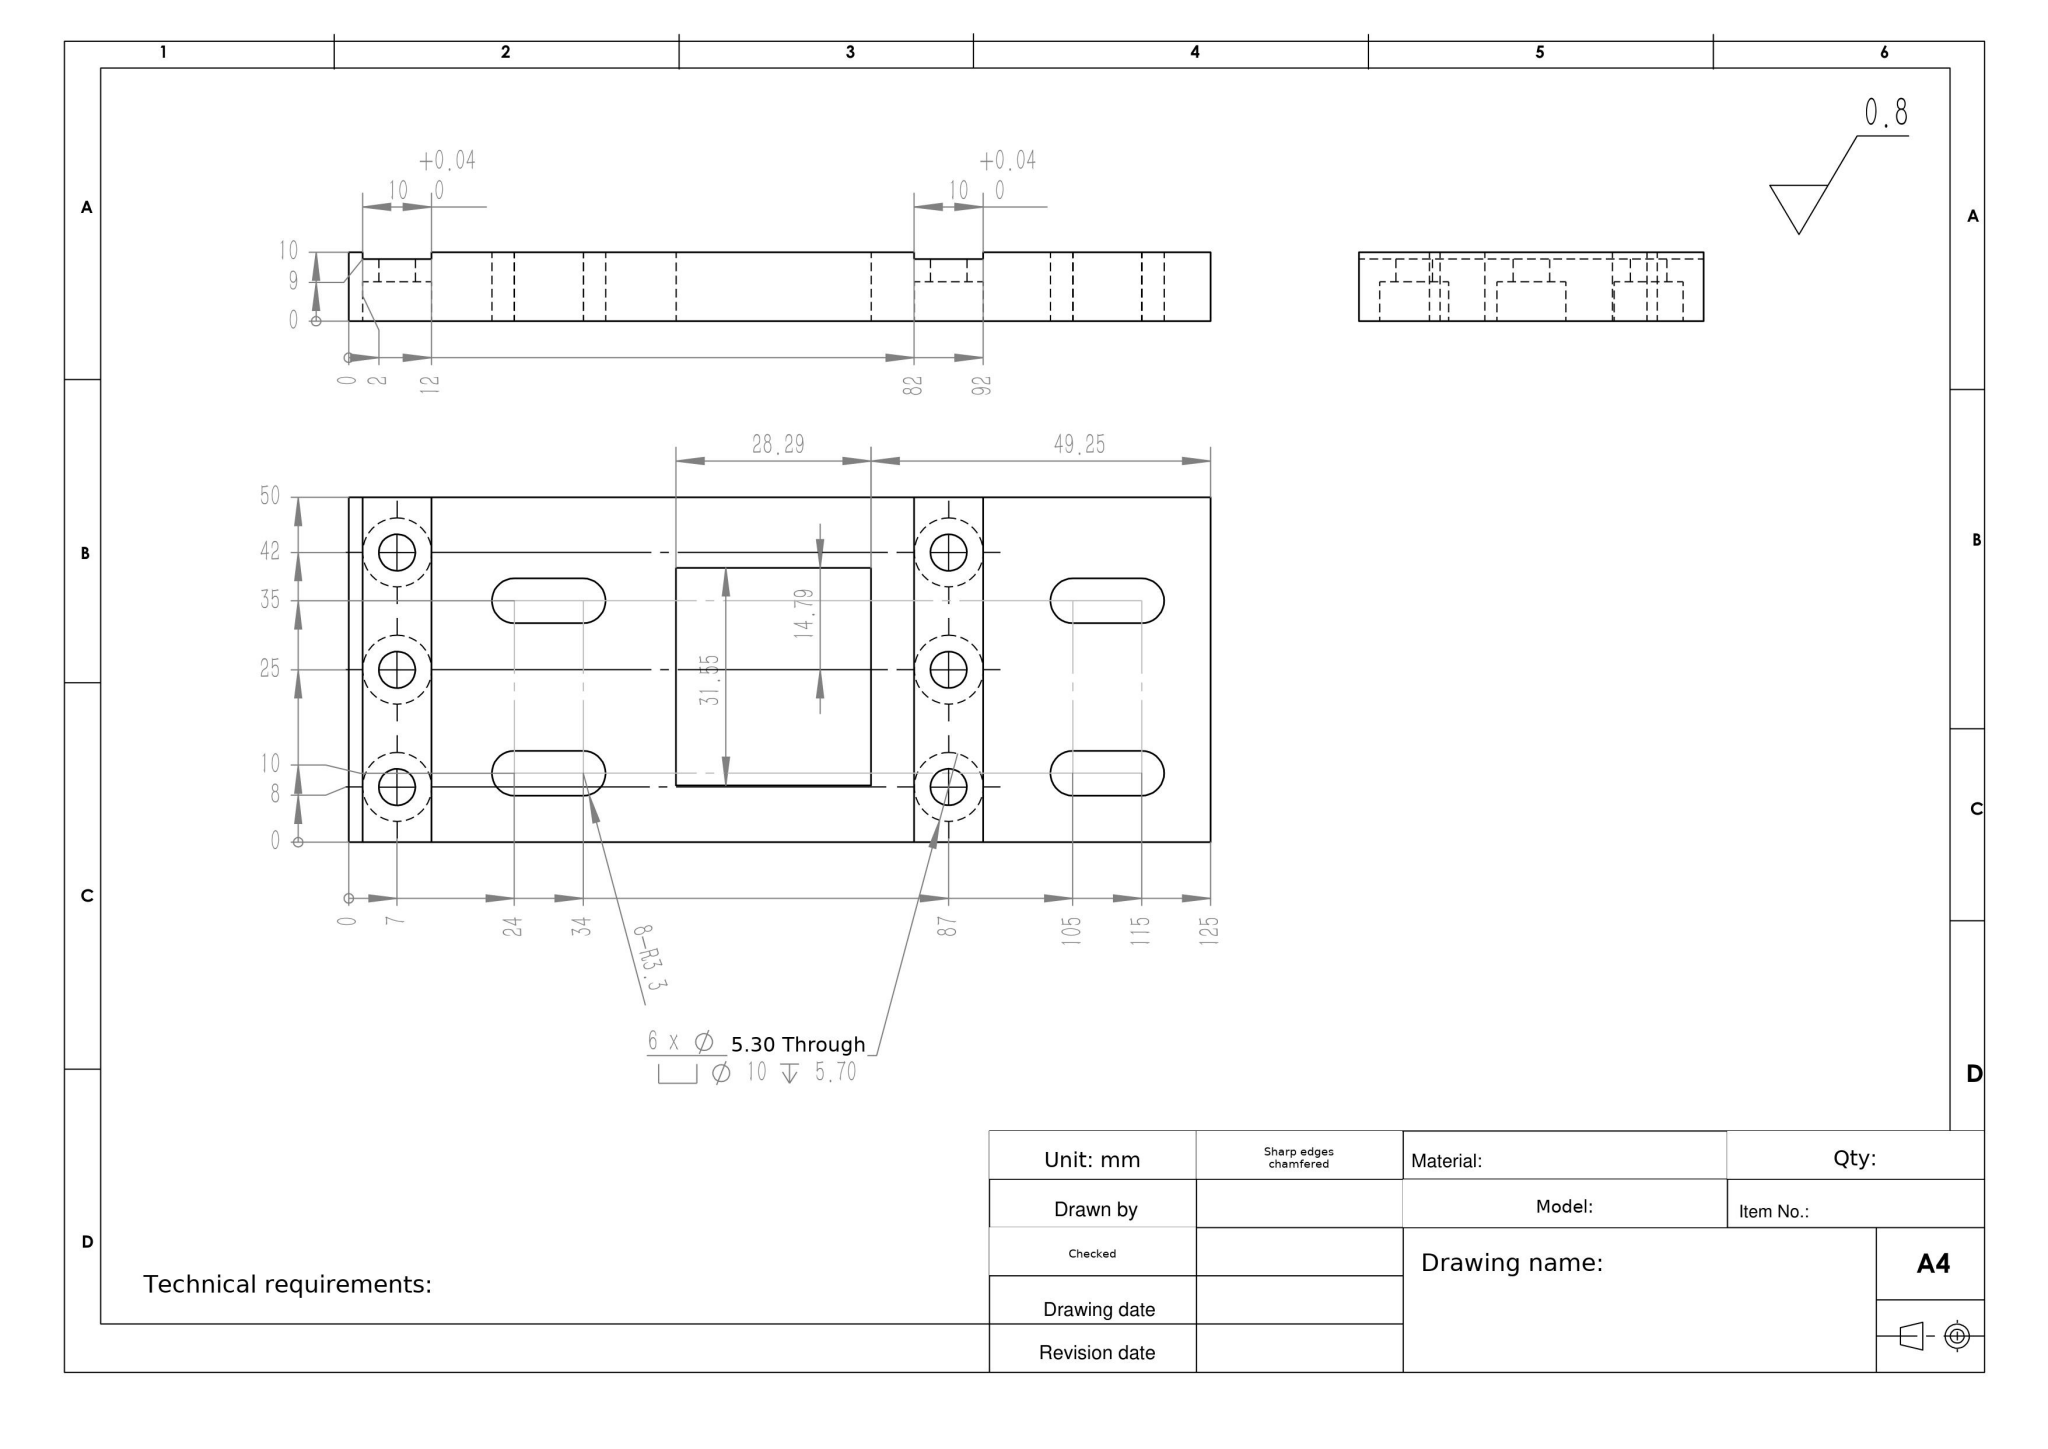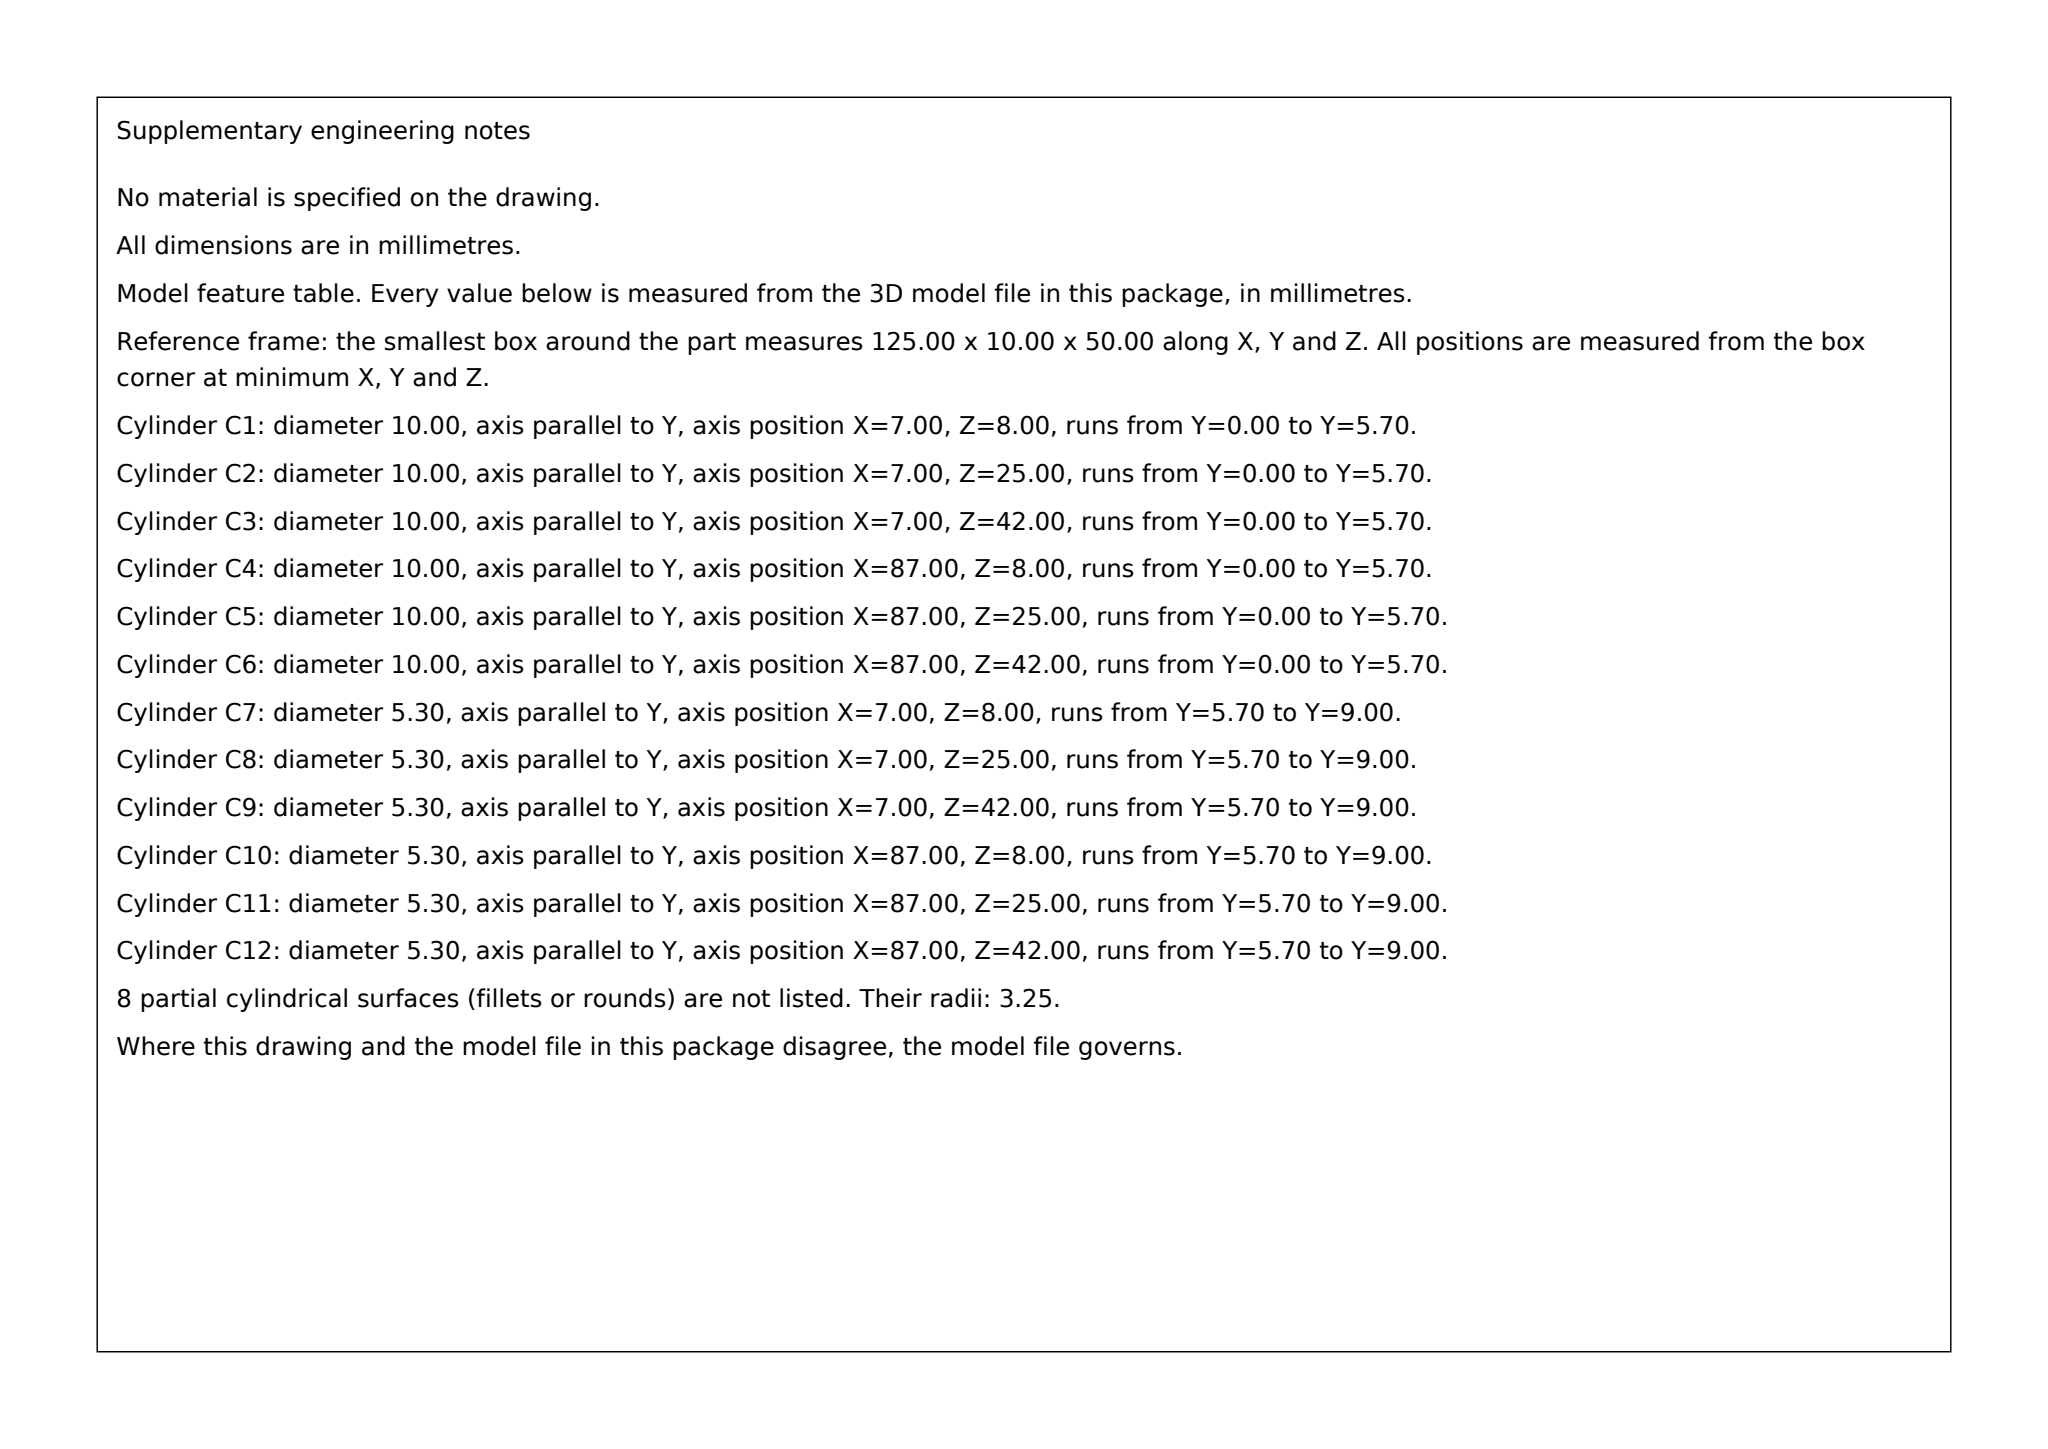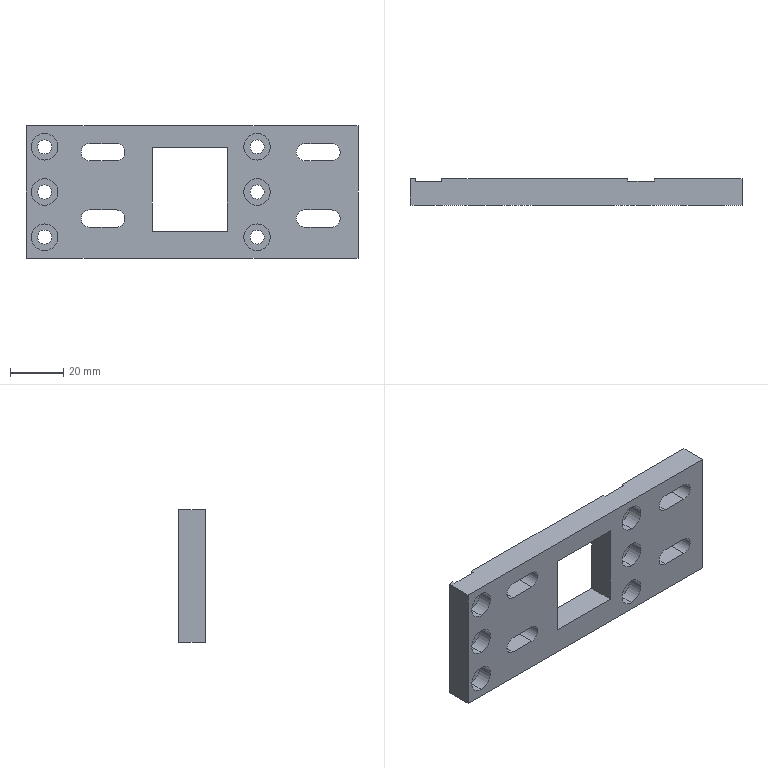Part | SolidWorks | mm | 1 solid | 68 faces | box 125 x 10 x 50 mm | volume 45524 mm3 | cylinder 36 | plane 32 | commonest cylinder face diameters 6.5 x12 10 x12 5.3 x12
build123d program:
from build123d import *

# Parameters (mm, degrees)
SKETCH1_W                                         = 125
SKETCH1_H                                         = 10
BOSS_EXTRUDE1_DEPTH                               = 50
SKETCH2_W                                         = 10
SKETCH2_H                                         = 1
CUT_EXTRUDE1_DEPTH                                = 136
HOLE_SIZE_ACCORDING_TO_HEXAGON_SOCKET_D           = 5.3
HOLE_SIZE_ACCORDING_TO_HEXAGON_SOCKET_CBORE_D     = 10
HOLE_SIZE_ACCORDING_TO_HEXAGON_SOCKET_CBORE_DEPTH = 5.7
CUT_EXTRUDE2_DEPTH                                = 136
SKETCH5_W                                         = 28.288
SKETCH5_H                                         = 31.552
CUT_EXTRUDE3_DEPTH                                = 33


with BuildPart() as part:
    # Sketch1 → Boss-Extrude1 (new body)
    with BuildSketch(Plane.XY):
        with Locations((62.5, 5)):
            Rectangle(SKETCH1_W, SKETCH1_H)
    extrude(amount=BOSS_EXTRUDE1_DEPTH)

    # Sketch2 → Cut-Extrude1 (cut, through all)
    with BuildSketch(Plane.XY.offset(50)):
        with Locations((7, 9.5)):
            Rectangle(SKETCH2_W, SKETCH2_H)
        with Locations((87, 9.5)):
            Rectangle(SKETCH2_W, SKETCH2_H)
    extrude(amount=-CUT_EXTRUDE1_DEPTH, mode=Mode.SUBTRACT)

    # Hole Size _According to_ Hexagon Socket (through all)
    with Locations(Plane(origin=(87, 0, 42), x_dir=(0, 0, -1), z_dir=(0, -1, 0))):
        with Locations((0, 0), (17, 0), (34, 0), (0, -80), (17, -80), (34, -80)):
            CounterBoreHole(HOLE_SIZE_ACCORDING_TO_HEXAGON_SOCKET_D / 2, HOLE_SIZE_ACCORDING_TO_HEXAGON_SOCKET_CBORE_D / 2, HOLE_SIZE_ACCORDING_TO_HEXAGON_SOCKET_CBORE_DEPTH)

    # Sketch4 → Cut-Extrude2 (cut, through all)
    with BuildSketch(Plane(origin=(0, 10, 0), x_dir=(1, 0, 0), z_dir=(0, 1, 0))):
        with BuildLine():
            Line((24, -11.75), (34, -11.75))
            ThreePointArc((34, -11.75), (37.25, -15), (34, -18.25))
            Line((34, -18.25), (24, -18.25))
            ThreePointArc((24, -18.25), (20.75, -15), (24, -11.75))
        make_face()
        with BuildLine():
            Line((24, -36.75), (34, -36.75))
            ThreePointArc((34, -36.75), (37.25, -40), (34, -43.25))
            Line((34, -43.25), (24, -43.25))
            ThreePointArc((24, -43.25), (20.75, -40), (24, -36.75))
        make_face()
        with BuildLine():
            Line((105, -11.75), (115, -11.75))
            ThreePointArc((115, -11.75), (118.25, -15), (115, -18.25))
            Line((115, -18.25), (105, -18.25))
            ThreePointArc((105, -18.25), (101.75, -15), (105, -11.75))
        make_face()
        with BuildLine():
            Line((105, -36.75), (115, -36.75))
            ThreePointArc((115, -36.75), (118.25, -40), (115, -43.25))
            Line((115, -43.25), (105, -43.25))
            ThreePointArc((105, -43.25), (101.75, -40), (105, -36.75))
        make_face()
    extrude(amount=-CUT_EXTRUDE2_DEPTH, mode=Mode.SUBTRACT)

    # Sketch5 → Cut-Extrude3 (cut)
    with BuildSketch(Plane(origin=(0, 10, 0), x_dir=(1, 0, 0), z_dir=(0, 1, 0))):
        with Locations((61.61, -25.989)):
            Rectangle(SKETCH5_W, SKETCH5_H)
    extrude(amount=-CUT_EXTRUDE3_DEPTH, mode=Mode.SUBTRACT)


solid = part.part